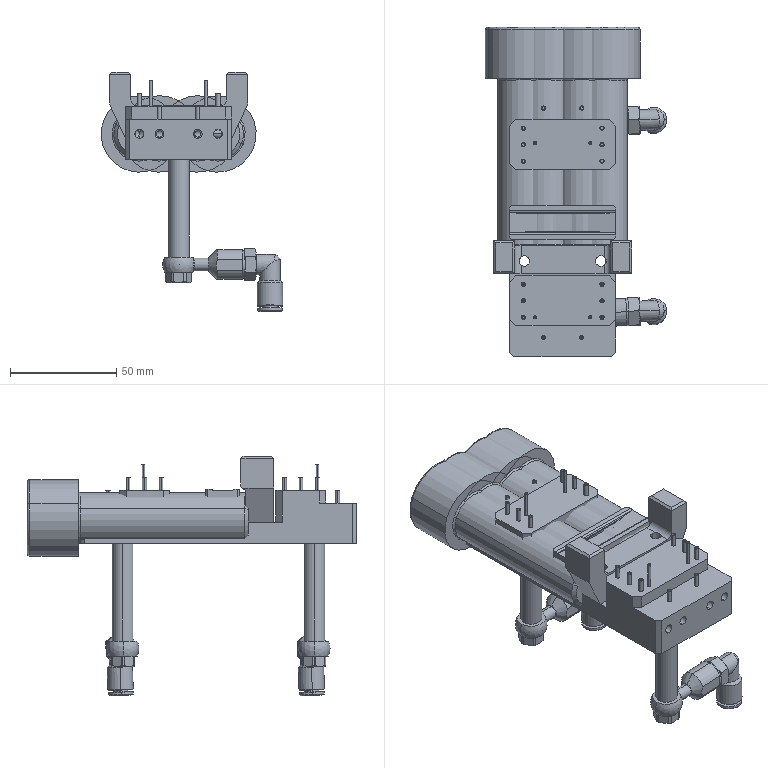Assembly | SolidWorks | mm | 23 component files | 43 solids | 1059 faces | box 85.49 x 155 x 112.66 mm | volume 370444 mm3 | cylinder 475 | plane 307 | cone 217 | torus 46 | spline 10 | sphere 4 | commonest cylinder face diameters 2 x68 1 x40 3 x38 6 x34 1.4 x32 4.2 x24 5 x24 10 x20
Bill of materials:
6.11-1937032103-0 | 1 | 45# | Rectangular base block with corner chamfers, two raised pads at the ends and a lower central channel between them; many small vertical pins stand up from the top faces, and holes run through the central floor and into the side faces.
6.11-1937032104-0 | 2 | Cr12MoV | Round flange with a long cylindrical shaft below it and a short stepped hub with a groove above it; a center bore runs through the hub, and the flange has three holes evenly spaced around it.
6.11-1937032105-0 | 1 | 45# | Solid rectangular bar with a long, shallow, curved groove along the top face and a smaller step or groove along one top edge; the top corners are chamfered or rounded.
6.11-1937032106-0 | 2 | 40Cr | Eye-shaped fitting body: a round eye with a through-hole and spherical-looking sides, joined by a narrow cylindrical neck and a conical transition to a larger hollow cylindrical cup.
6.11-1937032107-0 | 2 | 40Cr | Hexagonal base with a long cylindrical stem rising from it; the stem has a small bore at its tip and a chamfered end, and a small notch is visible near the bottom of the stem in one view.
6.11-1937032108-0 | 1 |  | U-shaped bracket block: a base with two upright end lugs, a flat floor between them with rounded inside corners, two through-holes in the floor, and tapered (angled) lower sides.
M5CopperSealingGasket | 4 | CopperT3 | Thin flat annular ring (washer-like disc) with a large central hole and plain flat faces.
M5SetScrew | 2 | 45 | Short solid cylinder with chamfered ends and a square-shaped recess (socket) in one end face; the other end is plain and flat.
NPB7 | 2 |  | Flat circular ring with a rectangular-looking cross-section and rounded or chamfered edges; the mesh surface is faceted.
NPQH-L-G18-Q6-P10 | 2 |  | 90-degree elbow body: one branch has a cylindrical stub, a hexagonal collar, and a cylindrical body ending in a rounded elbow; the other branch is a larger cylindrical sleeve ending in a narrow neck and a thin flange or collar.
socket head cap screw_iso | 4 |  | Headed pin or cap-screw-like part: a cylindrical head on a smaller-diameter plain cylindrical shank with a chamfered tip.
Mates:
1. coincident | 6.11-1937032103-0-1 face at (0, 45, 4) dir (0, 0, -1) | 6.11-1937032104-0-1 face at (0, 45, 4) dir (0, 0, 1)
2. concentric | 6.11-1937032103-0-1 face at (0, 45, 4) dir (0, 0, -1) r 16 | 6.11-1937032104-0-1 face at (0, 45, 0) dir (0, 0, 1) r 16
3. coincident | 6.11-1937032103-0-1 face at (0, -45, 4) dir (0, 0, -1) | 6.11-1937032104-0-2 face at (0, -45, 4) dir (0, 0, 1)
4. concentric | 6.11-1937032103-0-1 face at (0, -45, 4) dir (0, 0, -1) r 16 | 6.11-1937032104-0-2 face at (0, -45, 0) dir (0, 0, 1) r 16
5. parallel | 6.11-1937032103-0-1 face at (-25, 65, 25) dir (0, 1, 0) | 6.11-1937032104-0-1 plane at (0, 45, 4) dir (0, 1, 0)
6. coincident | 6.11-1937032103-0-1 face at (0, 0, 10) dir (0, 0, 1) | 6.11-1937032105-0-1 face at (0, -2, 10) dir (0, 0, -1)
7. coincident | 6.11-1937032103-0-1 face at (25, -65, 25) dir (1, 0, 0) | 6.11-1937032105-0-1 face at (25, 6, 28) dir (1, 0, 0)
8. concentric | 6.11-1937032103-0-1 face at (0, -55.5, 4) dir (0, 0, -1) r 1.65 | 6.11-1937032104-0-2 face at (0, -55.5, 0) dir (0, 0, -1) r 2.25
9. tangent | 6.11-1937032104-0-1 face at (0, 45, 6) dir (0, 0, 1) | NPB7-1 face at (-1.226, 48.385, 6.367) dir (1, 0, 0)
10. tangent | 6.11-1937032104-0-2 face at (0, -45, 6) dir (0, 0, 1) | NPB7-3 face at (-1.224, -41.615, 6.367) dir (1, 0, 0)
11. distance | 6.11-1937032105-0-1 face at (-25, 6, 28) dir (0, 1, 0) | 6.11-1937032103-0-1 face at (-25, 23, 10) dir (0, -1, 0)
12. concentric | 6.11-1937032104-0-1 face at (0, 45, -46) dir (0, 0, 1) r 5 | 6.11-1937032106-0-1 face at (0, 45, -53) dir (0, 0, -1) r 3
13. coincident | 6.11-1937032104-0-1 face at (0, 45, -46) dir (0, 0, -1) | 6.11-1937032106-0-1 face at (-7.088, 34.704, -46) dir (0, 0, 1)
14. coincident | 6.11-1937032106-0-1 face at (29.975, 46.218, -56.5) dir (0.9992, 0.0406, 0) | NPQH-L-G18-Q6-P10-1 face at (29.983, 46.017, -55.997) dir (-0.9992, -0.0406, 0)
15. concentric | 6.11-1937032106-0-1 face at (0, 45, -53) dir (0, 0, -1) r 3 | 6.11-1937032107-0-1 face at (0, 45, -35) dir (0, 0, -1) r 2.5
16. coincident | 6.11-1937032106-0-1 face at (-7.088, 34.704, -53) dir (0, 0, -1) | 6.11-1937032107-0-1 face at (0, 45, -53) dir (0, 0, 1)
17. coincident | 6.11-1937032106-0-2 face at (29.975, -43.782, -56.5) dir (0.9992, 0.0406, 0) | NPQH-L-G18-Q6-P10-2 face at (29.983, -43.983, -55.997) dir (-0.9992, -0.0406, 0)
18. concentric | 6.11-1937032106-0-2 face at (0, -45, -53) dir (0, 0, -1) r 3 | 6.11-1937032107-0-2 face at (0, -45, -35) dir (0, 0, -1) r 2.5
19. coincident | 6.11-1937032106-0-2 face at (-7.088, -55.296, -53) dir (0, 0, -1) | 6.11-1937032107-0-2 face at (0, -45, -53) dir (0, 0, 1)
20. concentric | 6.11-1937032104-0-2 face at (0, -45, -46) dir (0, 0, 1) r 5 | 6.11-1937032106-0-2 face at (0, -45, -53) dir (0, 0, -1) r 3
21. coincident | 6.11-1937032104-0-2 face at (0, -45, -46) dir (0, 0, -1) | 6.11-1937032106-0-2 face at (-7.088, -55.296, -46) dir (0, 0, 1)
22. coincident | 6.11-1937032103-0-1 face at (0, 0, 10) dir (0, 0, 1) | 6.11-1937032108-0-1 face at (-32.5, -26, 10) dir (0, 0, -1)
23. coincident | 6.11-1937032103-0-1 face at (0, 0, 10) dir (0, 0, 1) | 6.11-1937032108-0-1 face at (-32.5, -26, 10) dir (0, 0, -1)
24. distance | 6.11-1937032103-0-1 face at (-25, -27, 10) dir (0, 1, 0) | 6.11-1937032108-0-1 face at (0, -26, 25.5) dir (0, -1, 0)
25. width | 6.11-1937032108-0-1 face at (-32.5, -26, 41) dir (-1, 0, 0) | 6.11-1937032108-0-1 face at (32.5, -26, 41) dir (1, 0, 0) | 6.11-1937032103-0-1 face at (-25, -65, 25) dir (-1, 0, 0) | 6.11-1937032103-0-1 face at (25, -65, 25) dir (1, 0, 0)
26. concentric | socket head cap screw_iso-1 face at (18.5, 121.75, 12) dir (0, 1, 0) r 12 | 6.11-1937032103-0-1 face at (18.5, 65, 12) dir (0, 1, 0) r 2.1
27. distance | socket head cap screw_iso-1 face at (25.371, 66, 28.637) dir (0, -1, 0) | 6.11-1937032103-0-1 face at (-25, 65, 25) dir (0, 1, 0)
28. concentric | 6.11-1937032103-0-1 face at (9, 65, 12) dir (0, 1, 0) r 2.1 | socket head cap screw_iso-2 face at (9, 121.75, 12) dir (0, 1, 0) r 12
29. distance | socket head cap screw_iso-2 face at (15.871, 66, 28.637) dir (0, -1, 0) | 6.11-1937032103-0-1 face at (-25, 65, 25) dir (0, 1, 0)
30. concentric | 6.11-1937032103-0-1 face at (-9, 65, 12) dir (0, 1, 0) r 2.1 | socket head cap screw_iso-3 face at (-9, 121.75, 12) dir (0, 1, 0) r 12
31. distance | socket head cap screw_iso-3 face at (-2.129, 66, 28.637) dir (0, -1, 0) | 6.11-1937032103-0-1 face at (-25, 65, 25) dir (0, 1, 0)
32. concentric | 6.11-1937032103-0-1 face at (-18.5, 65, 12) dir (0, 1, 0) r 2.1 | socket head cap screw_iso-4 face at (-18.5, 121.75, 12) dir (0, 1, 0) r 12
33. distance | socket head cap screw_iso-4 face at (-11.629, 66, 28.637) dir (0, -1, 0) | 6.11-1937032103-0-1 face at (-25, 65, 25) dir (0, 1, 0)
34. coincident | 6.11-1937032103-0-1 face at (-25, 65, 25) dir (0, 1, 0) | M5CopperSealingGasket-1 face at (-18.5, 65, 12) dir (0, -1, 0)
35. concentric | 6.11-1937032103-0-1 face at (-18.5, 65, 12) dir (0, 1, 0) r 2.1 | M5CopperSealingGasket-1 face at (-18.5, 66, 12) dir (0, -1, 0) r 4.5
36. coincident | 6.11-1937032103-0-1 face at (-25, 65, 25) dir (0, 1, 0) | M5CopperSealingGasket-2 face at (-9, 65, 12) dir (0, -1, 0)
37. concentric | 6.11-1937032103-0-1 face at (-9, 65, 12) dir (0, 1, 0) r 2.1 | M5CopperSealingGasket-2 face at (-9, 66, 12) dir (0, -1, 0) r 4.5
38. coincident | 6.11-1937032103-0-1 face at (-25, 65, 25) dir (0, 1, 0) | M5CopperSealingGasket-3 face at (9, 65, 12) dir (0, -1, 0)
39. concentric | 6.11-1937032103-0-1 face at (9, 65, 12) dir (0, 1, 0) r 2.1 | M5CopperSealingGasket-3 face at (9, 66, 12) dir (0, -1, 0) r 4.5
40. coincident | 6.11-1937032103-0-1 face at (-25, 65, 25) dir (0, 1, 0) | M5CopperSealingGasket-4 face at (18.5, 65, 12) dir (0, -1, 0)
41. concentric | 6.11-1937032103-0-1 face at (18.5, 65, 12) dir (0, 1, 0) r 2.1 | M5CopperSealingGasket-4 face at (18.5, 66, 12) dir (0, -1, 0) r 4.5
42. concentric | 6.11-1937032103-0-1 face at (25, -46.5, 12) dir (1, 0, 0) r 2.1 | M5SetScrew-1 face at (25, -46.5, 12) dir (-1, 0, 0) r 2.1
43. coincident | 6.11-1937032103-0-1 face at (25, -65, 25) dir (1, 0, 0) | M5SetScrew-1 face at (25, -46.5, 12) dir (1, 0, 0)
44. concentric | 6.11-1937032103-0-1 face at (25, 47, 12) dir (1, 0, 0) r 2.1 | M5SetScrew-2 face at (25, 47, 12) dir (-1, 0, 0) r 2.1
45. coincident | 6.11-1937032103-0-1 face at (25, -65, 25) dir (1, 0, 0) | M5SetScrew-2 face at (25, 47, 12) dir (1, 0, 0)
46. concentric | 6.11-1937032104-0-1 face at (0, 45, 12) dir (0, 0, -1) r 5 | NPB7-1 face at (0, 45, 4.95) dir (0, 0, 1) r 5
47. concentric | 6.11-1937032104-0-2 face at (0, -45, 12) dir (0, 0, -1) r 5 | NPB7-3 face at (0, -45, 4.95) dir (0, 0, 1) r 5
48. concentric | 6.11-1937032106-0-1 face at (29.975, 46.218, -49.5) dir (0.9992, 0.0406, 0) r 4.4 | NPQH-L-G18-Q6-P10-1 face at (29.975, 46.218, -49.5) dir (-0.9992, -0.0406, 0) r 4.4
49. concentric | 6.11-1937032106-0-2 face at (29.975, -43.782, -49.5) dir (0.9992, 0.0406, 0) r 4.4 | NPQH-L-G18-Q6-P10-2 face at (29.975, -43.782, -49.5) dir (-0.9992, -0.0406, 0) r 4.4